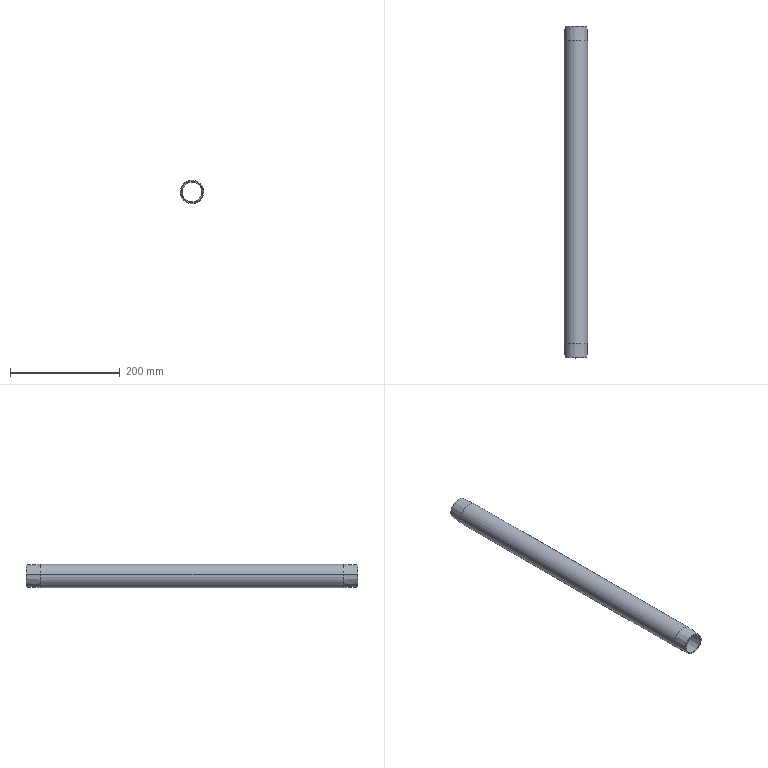Component | SolidWorks | YC1-250-04BalancerAssembly#16673-1_YC1-250-04-11Standpipe#16673-1 | 1 solid | 14 faces | box 42.7 x 604 x 42.7 mm | volume 154183 mm3 | cone 8 | cylinder 4 | plane 2 | commonest cylinder face diameters 42.7 x2 38.695 x2 | material Plain Carbon Steel
STEP:
#1=COLOUR_RGB('',0.7922,0.8196,0.9333);
#2=FILL_AREA_STYLE_COLOUR('',#1);
#3=FILL_AREA_STYLE('',(#2));
#4=SURFACE_STYLE_FILL_AREA(#3);
#5=SURFACE_SIDE_STYLE('',(#4));
#6=SURFACE_STYLE_USAGE(.BOTH.,#5);
#7=PRESENTATION_STYLE_ASSIGNMENT((#6));
#8=CARTESIAN_POINT('',(-18.941,180.098,-9.378));
#9=VERTEX_POINT('',#8);
#10=CARTESIAN_POINT('',(-17.28,180.098,-9.638));
#11=VERTEX_POINT('',#10);
#12=CARTESIAN_POINT('',(-18.11,180.098,-9.508));
#13=DIRECTION('',(-0.,-1.,0.));
#14=DIRECTION('',(-0.988,0.,0.1543));
#15=AXIS2_PLACEMENT_3D('',#12,#13,#14);
#16=CIRCLE('',#15,0.8406);
#17=EDGE_CURVE('',#9,#11,#16,.T.);
#18=ORIENTED_EDGE('',*,*,#17,.T.);
#19=CARTESIAN_POINT('',(-17.28,158.445,-9.638));
#20=VERTEX_POINT('',#19);
#21=CARTESIAN_POINT('',(-17.28,157.382,-9.638));
#22=DIRECTION('',(-0.,-1.,0.));
#23=VECTOR('',#22,39.37);
#24=LINE('',#21,#23);
#25=EDGE_CURVE('',#11,#20,#24,.T.);
#26=ORIENTED_EDGE('',*,*,#25,.T.);
#27=CARTESIAN_POINT('',(-18.941,158.445,-9.378));
#28=VERTEX_POINT('',#27);
#29=CARTESIAN_POINT('',(-18.11,158.445,-9.508));
#30=DIRECTION('',(0.,1.,-0.));
#31=DIRECTION('',(-0.988,0.,0.1543));
#32=AXIS2_PLACEMENT_3D('',#29,#30,#31);
#33=CIRCLE('',#32,0.8406);
#34=EDGE_CURVE('',#20,#28,#33,.T.);
#35=ORIENTED_EDGE('',*,*,#34,.T.);
#36=CARTESIAN_POINT('',(-18.941,157.382,-9.378));
#37=DIRECTION('',(-0.,-1.,0.));
#38=VECTOR('',#37,39.37);
#39=LINE('',#36,#38);
#40=EDGE_CURVE('',#9,#28,#39,.T.);
#41=ORIENTED_EDGE('',*,*,#40,.F.);
#42=EDGE_LOOP('',(#18,#26,#35,#41));
#43=FACE_OUTER_BOUND('',#42,.T.);
#44=CARTESIAN_POINT('',(-18.11,157.382,-9.508));
#45=DIRECTION('',(-0.,-1.,0.));
#46=DIRECTION('',(-0.988,0.,0.1543));
#47=AXIS2_PLACEMENT_3D('',#44,#45,#46);
#48=CYLINDRICAL_SURFACE('',#47,0.8406);
#49=ADVANCED_FACE('',(#43),#48,.T.);
#50=CARTESIAN_POINT('',(-17.332,157.382,-9.629));
#51=VERTEX_POINT('',#50);
#52=CARTESIAN_POINT('',(-18.888,157.382,-9.386));
#53=VERTEX_POINT('',#52);
#54=CARTESIAN_POINT('',(-18.11,157.382,-9.508));
#55=DIRECTION('',(0.,1.,-0.));
#56=DIRECTION('',(0.988,0.,-0.1543));
#57=AXIS2_PLACEMENT_3D('',#54,#55,#56);
#58=CIRCLE('',#57,0.7874);
#59=EDGE_CURVE('',#51,#53,#58,.T.);
#60=ORIENTED_EDGE('',*,*,#59,.T.);
#61=CARTESIAN_POINT('',(-18.941,158.445,-9.378));
#62=DIRECTION('',(-0.04934,0.9988,0.007708));
#63=VECTOR('',#62,39.37);
#64=LINE('',#61,#63);
#65=EDGE_CURVE('',#53,#28,#64,.T.);
#66=ORIENTED_EDGE('',*,*,#65,.T.);
#67=ORIENTED_EDGE('',*,*,#34,.F.);
#68=CARTESIAN_POINT('',(-17.28,158.445,-9.638));
#69=DIRECTION('',(0.04934,0.9988,-0.007708));
#70=VECTOR('',#69,39.37);
#71=LINE('',#68,#70);
#72=EDGE_CURVE('',#51,#20,#71,.T.);
#73=ORIENTED_EDGE('',*,*,#72,.F.);
#74=EDGE_LOOP('',(#60,#66,#67,#73));
#75=FACE_OUTER_BOUND('',#74,.T.);
#76=CARTESIAN_POINT('',(-18.11,158.445,-9.508));
#77=DIRECTION('',(0.,1.,-0.));
#78=DIRECTION('',(0.988,0.,-0.1543));
#79=AXIS2_PLACEMENT_3D('',#76,#77,#78);
#80=CONICAL_SURFACE('',#79,0.8406,0.04996);
#81=ADVANCED_FACE('',(#75),#80,.T.);
#82=CARTESIAN_POINT('',(-18.888,181.161,-9.386));
#83=VERTEX_POINT('',#82);
#84=CARTESIAN_POINT('',(-17.332,181.161,-9.629));
#85=VERTEX_POINT('',#84);
#86=CARTESIAN_POINT('',(-18.11,181.161,-9.508));
#87=DIRECTION('',(-0.,-1.,0.));
#88=DIRECTION('',(-0.988,0.,0.1543));
#89=AXIS2_PLACEMENT_3D('',#86,#87,#88);
#90=CIRCLE('',#89,0.7874);
#91=EDGE_CURVE('',#83,#85,#90,.T.);
#92=ORIENTED_EDGE('',*,*,#91,.T.);
#93=CARTESIAN_POINT('',(-17.28,180.098,-9.638));
#94=DIRECTION('',(0.04934,-0.9988,-0.007708));
#95=VECTOR('',#94,39.37);
#96=LINE('',#93,#95);
#97=EDGE_CURVE('',#85,#11,#96,.T.);
#98=ORIENTED_EDGE('',*,*,#97,.T.);
#99=ORIENTED_EDGE('',*,*,#17,.F.);
#100=CARTESIAN_POINT('',(-18.941,180.098,-9.378));
#101=DIRECTION('',(-0.04934,-0.9988,0.007708));
#102=VECTOR('',#101,39.37);
#103=LINE('',#100,#102);
#104=EDGE_CURVE('',#83,#9,#103,.T.);
#105=ORIENTED_EDGE('',*,*,#104,.F.);
#106=EDGE_LOOP('',(#92,#98,#99,#105));
#107=FACE_OUTER_BOUND('',#106,.T.);
#108=CARTESIAN_POINT('',(-18.11,180.098,-9.508));
#109=DIRECTION('',(-0.,-1.,0.));
#110=DIRECTION('',(-0.988,0.,0.1543));
#111=AXIS2_PLACEMENT_3D('',#108,#109,#110);
#112=CONICAL_SURFACE('',#111,0.8406,0.04996);
#113=ADVANCED_FACE('',(#107),#112,.T.);
#114=CARTESIAN_POINT('',(-17.41,157.382,-9.617));
#115=VERTEX_POINT('',#114);
#116=CARTESIAN_POINT('',(-18.81,157.382,-9.399));
#117=VERTEX_POINT('',#116);
#118=CARTESIAN_POINT('',(-18.11,157.382,-9.508));
#119=DIRECTION('',(-0.,-1.,0.));
#120=DIRECTION('',(0.988,0.,-0.1543));
#121=AXIS2_PLACEMENT_3D('',#118,#119,#120);
#122=CIRCLE('',#121,0.7086);
#123=EDGE_CURVE('',#115,#117,#122,.T.);
#124=ORIENTED_EDGE('',*,*,#123,.T.);
#125=CARTESIAN_POINT('',(-18.863,158.445,-9.39));
#126=VERTEX_POINT('',#125);
#127=CARTESIAN_POINT('',(-18.863,158.445,-9.39));
#128=DIRECTION('',(-0.04934,0.9988,0.007708));
#129=VECTOR('',#128,39.37);
#130=LINE('',#127,#129);
#131=EDGE_CURVE('',#117,#126,#130,.T.);
#132=ORIENTED_EDGE('',*,*,#131,.T.);
#133=CARTESIAN_POINT('',(-17.358,158.445,-9.625));
#134=VERTEX_POINT('',#133);
#135=CARTESIAN_POINT('',(-18.11,158.445,-9.508));
#136=DIRECTION('',(-0.,-1.,0.));
#137=DIRECTION('',(0.988,0.,-0.1543));
#138=AXIS2_PLACEMENT_3D('',#135,#136,#137);
#139=CIRCLE('',#138,0.7617);
#140=EDGE_CURVE('',#134,#126,#139,.T.);
#141=ORIENTED_EDGE('',*,*,#140,.F.);
#142=CARTESIAN_POINT('',(-17.358,158.445,-9.625));
#143=DIRECTION('',(0.04934,0.9988,-0.007708));
#144=VECTOR('',#143,39.37);
#145=LINE('',#142,#144);
#146=EDGE_CURVE('',#115,#134,#145,.T.);
#147=ORIENTED_EDGE('',*,*,#146,.F.);
#148=EDGE_LOOP('',(#124,#132,#141,#147));
#149=FACE_OUTER_BOUND('',#148,.T.);
#150=CARTESIAN_POINT('',(-18.11,158.445,-9.508));
#151=DIRECTION('',(0.,1.,-0.));
#152=DIRECTION('',(0.988,0.,-0.1543));
#153=AXIS2_PLACEMENT_3D('',#150,#151,#152);
#154=CONICAL_SURFACE('',#153,0.7617,0.04996);
#155=ADVANCED_FACE('',(#149),#154,.F.);
#156=CARTESIAN_POINT('',(-18.81,181.161,-9.399));
#157=VERTEX_POINT('',#156);
#158=CARTESIAN_POINT('',(-17.41,181.161,-9.617));
#159=VERTEX_POINT('',#158);
#160=CARTESIAN_POINT('',(-18.11,181.161,-9.508));
#161=DIRECTION('',(0.,1.,-0.));
#162=DIRECTION('',(-0.988,0.,0.1543));
#163=AXIS2_PLACEMENT_3D('',#160,#161,#162);
#164=CIRCLE('',#163,0.7086);
#165=EDGE_CURVE('',#157,#159,#164,.T.);
#166=ORIENTED_EDGE('',*,*,#165,.T.);
#167=CARTESIAN_POINT('',(-17.358,180.098,-9.625));
#168=VERTEX_POINT('',#167);
#169=CARTESIAN_POINT('',(-17.358,180.098,-9.625));
#170=DIRECTION('',(0.04934,-0.9988,-0.007708));
#171=VECTOR('',#170,39.37);
#172=LINE('',#169,#171);
#173=EDGE_CURVE('',#159,#168,#172,.T.);
#174=ORIENTED_EDGE('',*,*,#173,.T.);
#175=CARTESIAN_POINT('',(-18.863,180.098,-9.39));
#176=VERTEX_POINT('',#175);
#177=CARTESIAN_POINT('',(-18.11,180.098,-9.508));
#178=DIRECTION('',(0.,1.,-0.));
#179=DIRECTION('',(-0.988,0.,0.1543));
#180=AXIS2_PLACEMENT_3D('',#177,#178,#179);
#181=CIRCLE('',#180,0.7617);
#182=EDGE_CURVE('',#176,#168,#181,.T.);
#183=ORIENTED_EDGE('',*,*,#182,.F.);
#184=CARTESIAN_POINT('',(-18.863,180.098,-9.39));
#185=DIRECTION('',(-0.04934,-0.9988,0.007708));
#186=VECTOR('',#185,39.37);
#187=LINE('',#184,#186);
#188=EDGE_CURVE('',#157,#176,#187,.T.);
#189=ORIENTED_EDGE('',*,*,#188,.F.);
#190=EDGE_LOOP('',(#166,#174,#183,#189));
#191=FACE_OUTER_BOUND('',#190,.T.);
#192=CARTESIAN_POINT('',(-18.11,180.098,-9.508));
#193=DIRECTION('',(-0.,-1.,0.));
#194=DIRECTION('',(-0.988,0.,0.1543));
#195=AXIS2_PLACEMENT_3D('',#192,#193,#194);
#196=CONICAL_SURFACE('',#195,0.7617,0.04996);
#197=ADVANCED_FACE('',(#191),#196,.F.);
#198=ORIENTED_EDGE('',*,*,#182,.T.);
#199=CARTESIAN_POINT('',(-17.358,157.382,-9.625));
#200=DIRECTION('',(-0.,-1.,0.));
#201=VECTOR('',#200,39.37);
#202=LINE('',#199,#201);
#203=EDGE_CURVE('',#168,#134,#202,.T.);
#204=ORIENTED_EDGE('',*,*,#203,.T.);
#205=ORIENTED_EDGE('',*,*,#140,.T.);
#206=CARTESIAN_POINT('',(-18.863,157.382,-9.39));
#207=DIRECTION('',(-0.,-1.,0.));
#208=VECTOR('',#207,39.37);
#209=LINE('',#206,#208);
#210=EDGE_CURVE('',#176,#126,#209,.T.);
#211=ORIENTED_EDGE('',*,*,#210,.F.);
#212=EDGE_LOOP('',(#198,#204,#205,#211));
#213=FACE_OUTER_BOUND('',#212,.T.);
#214=CARTESIAN_POINT('',(-18.11,157.382,-9.508));
#215=DIRECTION('',(-0.,-1.,0.));
#216=DIRECTION('',(-0.988,0.,0.1543));
#217=AXIS2_PLACEMENT_3D('',#214,#215,#216);
#218=CYLINDRICAL_SURFACE('',#217,0.7617);
#219=ADVANCED_FACE('',(#213),#218,.F.);
#220=ORIENTED_EDGE('',*,*,#25,.F.);
#221=CARTESIAN_POINT('',(-18.11,180.098,-9.508));
#222=DIRECTION('',(-0.,-1.,0.));
#223=DIRECTION('',(-0.988,0.,0.1543));
#224=AXIS2_PLACEMENT_3D('',#221,#222,#223);
#225=CIRCLE('',#224,0.8406);
#226=EDGE_CURVE('',#11,#9,#225,.T.);
#227=ORIENTED_EDGE('',*,*,#226,.T.);
#228=ORIENTED_EDGE('',*,*,#40,.T.);
#229=CARTESIAN_POINT('',(-18.11,158.445,-9.508));
#230=DIRECTION('',(0.,1.,-0.));
#231=DIRECTION('',(-0.988,0.,0.1543));
#232=AXIS2_PLACEMENT_3D('',#229,#230,#231);
#233=CIRCLE('',#232,0.8406);
#234=EDGE_CURVE('',#28,#20,#233,.T.);
#235=ORIENTED_EDGE('',*,*,#234,.T.);
#236=EDGE_LOOP('',(#220,#227,#228,#235));
#237=FACE_OUTER_BOUND('',#236,.T.);
#238=CARTESIAN_POINT('',(-18.11,157.382,-9.508));
#239=DIRECTION('',(-0.,-1.,0.));
#240=DIRECTION('',(-0.988,0.,0.1543));
#241=AXIS2_PLACEMENT_3D('',#238,#239,#240);
#242=CYLINDRICAL_SURFACE('',#241,0.8406);
#243=ADVANCED_FACE('',(#237),#242,.T.);
#244=ORIENTED_EDGE('',*,*,#65,.F.);
#245=CARTESIAN_POINT('',(-18.11,157.382,-9.508));
#246=DIRECTION('',(0.,1.,-0.));
#247=DIRECTION('',(0.988,0.,-0.1543));
#248=AXIS2_PLACEMENT_3D('',#245,#246,#247);
#249=CIRCLE('',#248,0.7874);
#250=EDGE_CURVE('',#53,#51,#249,.T.);
#251=ORIENTED_EDGE('',*,*,#250,.T.);
#252=ORIENTED_EDGE('',*,*,#72,.T.);
#253=ORIENTED_EDGE('',*,*,#234,.F.);
#254=EDGE_LOOP('',(#244,#251,#252,#253));
#255=FACE_OUTER_BOUND('',#254,.T.);
#256=CARTESIAN_POINT('',(-18.11,158.445,-9.508));
#257=DIRECTION('',(0.,1.,-0.));
#258=DIRECTION('',(0.988,0.,-0.1543));
#259=AXIS2_PLACEMENT_3D('',#256,#257,#258);
#260=CONICAL_SURFACE('',#259,0.8406,0.04996);
#261=ADVANCED_FACE('',(#255),#260,.T.);
#262=ORIENTED_EDGE('',*,*,#97,.F.);
#263=CARTESIAN_POINT('',(-18.11,181.161,-9.508));
#264=DIRECTION('',(-0.,-1.,0.));
#265=DIRECTION('',(-0.988,0.,0.1543));
#266=AXIS2_PLACEMENT_3D('',#263,#264,#265);
#267=CIRCLE('',#266,0.7874);
#268=EDGE_CURVE('',#85,#83,#267,.T.);
#269=ORIENTED_EDGE('',*,*,#268,.T.);
#270=ORIENTED_EDGE('',*,*,#104,.T.);
#271=ORIENTED_EDGE('',*,*,#226,.F.);
#272=EDGE_LOOP('',(#262,#269,#270,#271));
#273=FACE_OUTER_BOUND('',#272,.T.);
#274=CARTESIAN_POINT('',(-18.11,180.098,-9.508));
#275=DIRECTION('',(-0.,-1.,0.));
#276=DIRECTION('',(-0.988,0.,0.1543));
#277=AXIS2_PLACEMENT_3D('',#274,#275,#276);
#278=CONICAL_SURFACE('',#277,0.8406,0.04996);
#279=ADVANCED_FACE('',(#273),#278,.T.);
#280=ORIENTED_EDGE('',*,*,#59,.F.);
#281=ORIENTED_EDGE('',*,*,#250,.F.);
#282=EDGE_LOOP('',(#280,#281));
#283=FACE_OUTER_BOUND('',#282,.T.);
#284=ORIENTED_EDGE('',*,*,#123,.F.);
#285=CARTESIAN_POINT('',(-18.11,157.382,-9.508));
#286=DIRECTION('',(-0.,-1.,0.));
#287=DIRECTION('',(0.988,0.,-0.1543));
#288=AXIS2_PLACEMENT_3D('',#285,#286,#287);
#289=CIRCLE('',#288,0.7086);
#290=EDGE_CURVE('',#117,#115,#289,.T.);
#291=ORIENTED_EDGE('',*,*,#290,.F.);
#292=EDGE_LOOP('',(#284,#291));
#293=FACE_BOUND('',#292,.T.);
#294=CARTESIAN_POINT('',(-17.989,157.382,-8.73));
#295=DIRECTION('',(0.,1.,-0.));
#296=DIRECTION('',(0.988,-0.,-0.1543));
#297=AXIS2_PLACEMENT_3D('',#294,#295,#296);
#298=PLANE('',#297);
#299=ADVANCED_FACE('',(#283,#293),#298,.F.);
#300=ORIENTED_EDGE('',*,*,#165,.F.);
#301=CARTESIAN_POINT('',(-18.11,181.161,-9.508));
#302=DIRECTION('',(0.,1.,-0.));
#303=DIRECTION('',(-0.988,0.,0.1543));
#304=AXIS2_PLACEMENT_3D('',#301,#302,#303);
#305=CIRCLE('',#304,0.7086);
#306=EDGE_CURVE('',#159,#157,#305,.T.);
#307=ORIENTED_EDGE('',*,*,#306,.F.);
#308=EDGE_LOOP('',(#300,#307));
#309=FACE_BOUND('',#308,.T.);
#310=ORIENTED_EDGE('',*,*,#91,.F.);
#311=ORIENTED_EDGE('',*,*,#268,.F.);
#312=EDGE_LOOP('',(#310,#311));
#313=FACE_OUTER_BOUND('',#312,.T.);
#314=CARTESIAN_POINT('',(-17.989,181.161,-8.73));
#315=DIRECTION('',(-0.,-1.,0.));
#316=DIRECTION('',(-0.988,0.,0.1543));
#317=AXIS2_PLACEMENT_3D('',#314,#315,#316);
#318=PLANE('',#317);
#319=ADVANCED_FACE('',(#309,#313),#318,.F.);
#320=ORIENTED_EDGE('',*,*,#131,.F.);
#321=ORIENTED_EDGE('',*,*,#290,.T.);
#322=ORIENTED_EDGE('',*,*,#146,.T.);
#323=CARTESIAN_POINT('',(-18.11,158.445,-9.508));
#324=DIRECTION('',(-0.,-1.,0.));
#325=DIRECTION('',(0.988,0.,-0.1543));
#326=AXIS2_PLACEMENT_3D('',#323,#324,#325);
#327=CIRCLE('',#326,0.7617);
#328=EDGE_CURVE('',#126,#134,#327,.T.);
#329=ORIENTED_EDGE('',*,*,#328,.F.);
#330=EDGE_LOOP('',(#320,#321,#322,#329));
#331=FACE_OUTER_BOUND('',#330,.T.);
#332=CARTESIAN_POINT('',(-18.11,158.445,-9.508));
#333=DIRECTION('',(0.,1.,-0.));
#334=DIRECTION('',(0.988,0.,-0.1543));
#335=AXIS2_PLACEMENT_3D('',#332,#333,#334);
#336=CONICAL_SURFACE('',#335,0.7617,0.04996);
#337=ADVANCED_FACE('',(#331),#336,.F.);
#338=ORIENTED_EDGE('',*,*,#173,.F.);
#339=ORIENTED_EDGE('',*,*,#306,.T.);
#340=ORIENTED_EDGE('',*,*,#188,.T.);
#341=CARTESIAN_POINT('',(-18.11,180.098,-9.508));
#342=DIRECTION('',(0.,1.,-0.));
#343=DIRECTION('',(-0.988,0.,0.1543));
#344=AXIS2_PLACEMENT_3D('',#341,#342,#343);
#345=CIRCLE('',#344,0.7617);
#346=EDGE_CURVE('',#168,#176,#345,.T.);
#347=ORIENTED_EDGE('',*,*,#346,.F.);
#348=EDGE_LOOP('',(#338,#339,#340,#347));
#349=FACE_OUTER_BOUND('',#348,.T.);
#350=CARTESIAN_POINT('',(-18.11,180.098,-9.508));
#351=DIRECTION('',(-0.,-1.,0.));
#352=DIRECTION('',(-0.988,0.,0.1543));
#353=AXIS2_PLACEMENT_3D('',#350,#351,#352);
#354=CONICAL_SURFACE('',#353,0.7617,0.04996);
#355=ADVANCED_FACE('',(#349),#354,.F.);
#356=ORIENTED_EDGE('',*,*,#203,.F.);
#357=ORIENTED_EDGE('',*,*,#346,.T.);
#358=ORIENTED_EDGE('',*,*,#210,.T.);
#359=ORIENTED_EDGE('',*,*,#328,.T.);
#360=EDGE_LOOP('',(#356,#357,#358,#359));
#361=FACE_OUTER_BOUND('',#360,.T.);
#362=CARTESIAN_POINT('',(-18.11,157.382,-9.508));
#363=DIRECTION('',(-0.,-1.,0.));
#364=DIRECTION('',(-0.988,0.,0.1543));
#365=AXIS2_PLACEMENT_3D('',#362,#363,#364);
#366=CYLINDRICAL_SURFACE('',#365,0.7617);
#367=ADVANCED_FACE('',(#361),#366,.F.);
#368=CLOSED_SHELL('',(#49,#81,#113,#155,#197,#219,#243,#261,#279,#299,#319,#337,#355,#367));
#369=MANIFOLD_SOLID_BREP('',#368);
#370=STYLED_ITEM('',(#7),#369);
#371=(LENGTH_UNIT()NAMED_UNIT(*)SI_UNIT($,.METRE.));
#372=LENGTH_MEASURE_WITH_UNIT(LENGTH_MEASURE(0.0254),#371);
#373=DIMENSIONAL_EXPONENTS(1.,0.,0.,0.,0.,0.,0.);
#374=(CONVERSION_BASED_UNIT('',#372)LENGTH_UNIT()NAMED_UNIT(#373));
#375=UNCERTAINTY_MEASURE_WITH_UNIT(LENGTH_MEASURE(0.00001),#374,'','');
#376=(NAMED_UNIT(*)PLANE_ANGLE_UNIT()SI_UNIT($,.RADIAN.));
#377=(NAMED_UNIT(*)SI_UNIT($,.STERADIAN.)SOLID_ANGLE_UNIT());
#378=(GEOMETRIC_REPRESENTATION_CONTEXT(3)GLOBAL_UNCERTAINTY_ASSIGNED_CONTEXT((#375))GLOBAL_UNIT_ASSIGNED_CONTEXT((#374,#376,#377))REPRESENTATION_CONTEXT('',''));
#379=MECHANICAL_DESIGN_GEOMETRIC_PRESENTATION_REPRESENTATION('',(#370),#378);
#380=PRESENTATION_LAYER_ASSIGNMENT('','',(#370));
#381=CARTESIAN_POINT('',(0.,0.,0.));
#382=DIRECTION('',(0.,0.,1.));
#383=DIRECTION('',(1.,0.,0.));
#384=AXIS2_PLACEMENT_3D('',#381,#382,#383);
#385=(LENGTH_UNIT()NAMED_UNIT(*)SI_UNIT($,.METRE.));
#386=LENGTH_MEASURE_WITH_UNIT(LENGTH_MEASURE(0.0254),#385);
#387=DIMENSIONAL_EXPONENTS(1.,0.,0.,0.,0.,0.,0.);
#388=(CONVERSION_BASED_UNIT('',#386)LENGTH_UNIT()NAMED_UNIT(#387));
#389=UNCERTAINTY_MEASURE_WITH_UNIT(LENGTH_MEASURE(0.00001),#388,'','');
#390=(NAMED_UNIT(*)PLANE_ANGLE_UNIT()SI_UNIT($,.RADIAN.));
#391=(NAMED_UNIT(*)SI_UNIT($,.STERADIAN.)SOLID_ANGLE_UNIT());
#392=(GEOMETRIC_REPRESENTATION_CONTEXT(3)GLOBAL_UNCERTAINTY_ASSIGNED_CONTEXT((#389))GLOBAL_UNIT_ASSIGNED_CONTEXT((#388,#390,#391))REPRESENTATION_CONTEXT('',''));
#393=ADVANCED_BREP_SHAPE_REPRESENTATION('',(#369,#384),#392);